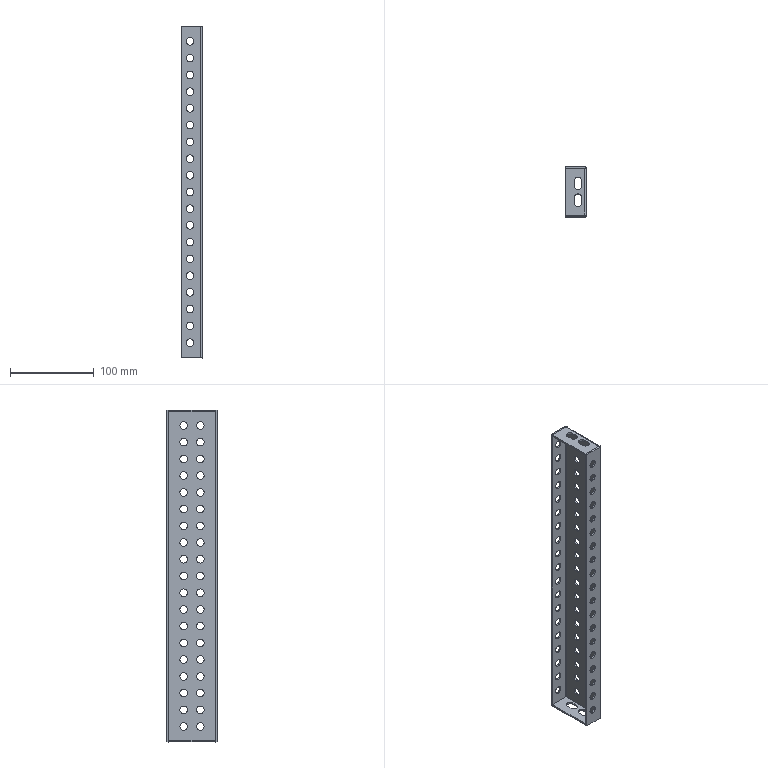Component | SolidWorks | KSHE-016.006-1 | 1 solid | 210 faces | volume 77832 mm3 | cylinder 168 | plane 42 | commonest cylinder face diameters 9 x160 4.2 x4 0.2 x4